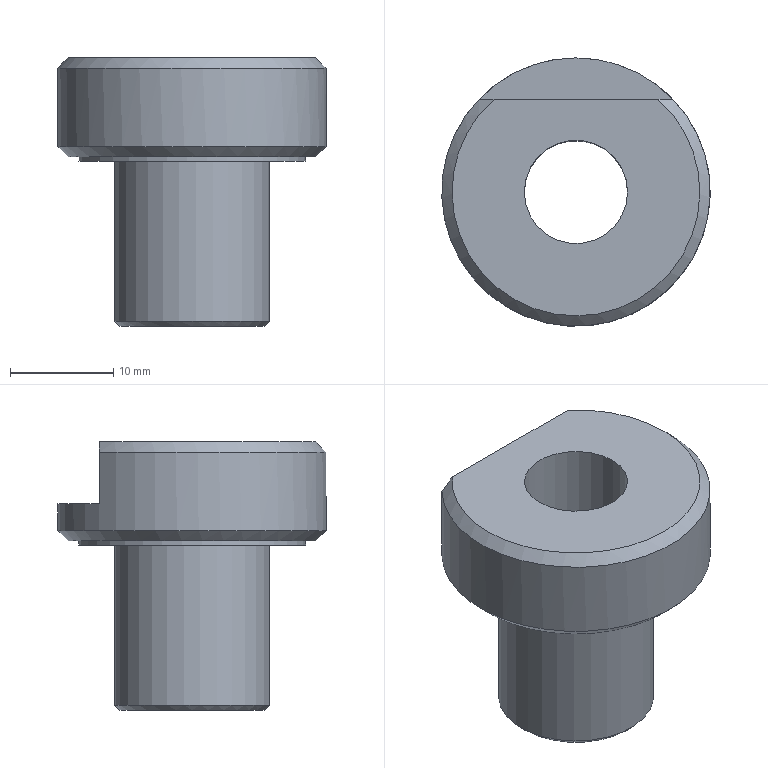Component | NX | DRILL_BUSHING | 1 solid | 13 faces | box 26 x 26 x 26 mm | volume 5648 mm3 | plane 6 | cylinder 4 | cone 3 | commonest cylinder face diameters 15 x1 22 x1 26 x1 10 x1
STEP:
#1=CARTESIAN_POINT('',(0.,0.,0.));
#2=DIRECTION('',(0.,0.,1.));
#3=DIRECTION('',(1.,0.,0.));
#4=AXIS2_PLACEMENT_3D('',#1,#2,#3);
#5=CARTESIAN_POINT('',(7.5,30.,-103.5));
#6=VERTEX_POINT('',#5);
#7=CARTESIAN_POINT('',(-0.,30.,-103.5));
#8=DIRECTION('',(0.,0.,1.));
#9=DIRECTION('',(1.,0.,0.));
#10=AXIS2_PLACEMENT_3D('',#7,#8,#9);
#11=CIRCLE('',#10,7.5);
#12=CARTESIAN_POINT('',(-0.,30.,-88.));
#13=DIRECTION('',(0.,0.,-1.));
#14=DIRECTION('',(-1.,0.,0.));
#15=AXIS2_PLACEMENT_3D('',#12,#13,#14);
#16=CYLINDRICAL_SURFACE('',#15,7.5);
#17=CARTESIAN_POINT('',(9.425,15.5));
#18=DIRECTION('',(-1.,0.));
#19=VECTOR('',#18,1.);
#20=LINE('',#17,#19);
#21=(GEOMETRIC_REPRESENTATION_CONTEXT(2)PARAMETRIC_REPRESENTATION_CONTEXT()REPRESENTATION_CONTEXT('',''));
#22=DEFINITIONAL_REPRESENTATION('',(#20),#21);
#23=PCURVE('',#16,#22);
#24=CARTESIAN_POINT('',(-0.,30.,-103.5));
#25=DIRECTION('',(0.,0.,1.));
#26=DIRECTION('',(1.,0.,0.));
#27=AXIS2_PLACEMENT_3D('',#24,#25,#26);
#28=CONICAL_SURFACE('',#27,7.5,0.7854);
#29=CARTESIAN_POINT('',(0.,0.));
#30=DIRECTION('',(1.,0.));
#31=VECTOR('',#30,1.);
#32=LINE('',#29,#31);
#33=(GEOMETRIC_REPRESENTATION_CONTEXT(2)PARAMETRIC_REPRESENTATION_CONTEXT()REPRESENTATION_CONTEXT('',''));
#34=DEFINITIONAL_REPRESENTATION('',(#32),#33);
#35=PCURVE('',#28,#34);
#36=SURFACE_CURVE('',#11,(#23,#35),.PCURVE_S1.);
#37=EDGE_CURVE('',#6,#6,#36,.T.);
#38=ORIENTED_EDGE('',*,*,#37,.T.);
#39=CARTESIAN_POINT('',(7.5,30.,-88.));
#40=VERTEX_POINT('',#39);
#41=CARTESIAN_POINT('',(7.5,30.,-88.));
#42=CARTESIAN_POINT('',(7.5,30.,-103.5));
#43=B_SPLINE_CURVE_WITH_KNOTS('',1,(#41,#42),.UNSPECIFIED.,.F.,.F.,(2,2),(0.,15.5),.PIECEWISE_BEZIER_KNOTS.);
#44=CARTESIAN_POINT('',(3.142,0.));
#45=DIRECTION('',(0.,1.));
#46=VECTOR('',#45,1.);
#47=LINE('',#44,#46);
#48=(GEOMETRIC_REPRESENTATION_CONTEXT(2)PARAMETRIC_REPRESENTATION_CONTEXT()REPRESENTATION_CONTEXT('',''));
#49=DEFINITIONAL_REPRESENTATION('',(#47),#48);
#50=PCURVE('',#16,#49);
#51=CARTESIAN_POINT('',(9.425,0.));
#52=DIRECTION('',(0.,1.));
#53=VECTOR('',#52,1.);
#54=LINE('',#51,#53);
#55=(GEOMETRIC_REPRESENTATION_CONTEXT(2)PARAMETRIC_REPRESENTATION_CONTEXT()REPRESENTATION_CONTEXT('',''));
#56=DEFINITIONAL_REPRESENTATION('',(#54),#55);
#57=PCURVE('',#16,#56);
#58=SEAM_CURVE('',#43,(#50,#57),.PCURVE_S1.);
#59=EDGE_CURVE('',#40,#6,#58,.T.);
#60=ORIENTED_EDGE('',*,*,#59,.F.);
#61=CARTESIAN_POINT('',(-0.,30.,-88.));
#62=DIRECTION('',(0.,0.,1.));
#63=DIRECTION('',(1.,0.,0.));
#64=AXIS2_PLACEMENT_3D('',#61,#62,#63);
#65=CIRCLE('',#64,7.5);
#66=CARTESIAN_POINT('',(9.425,0.));
#67=DIRECTION('',(-1.,0.));
#68=VECTOR('',#67,1.);
#69=LINE('',#66,#68);
#70=(GEOMETRIC_REPRESENTATION_CONTEXT(2)PARAMETRIC_REPRESENTATION_CONTEXT()REPRESENTATION_CONTEXT('',''));
#71=DEFINITIONAL_REPRESENTATION('',(#69),#70);
#72=PCURVE('',#16,#71);
#73=CARTESIAN_POINT('',(-0.,30.,-88.));
#74=DIRECTION('',(0.,0.,1.));
#75=DIRECTION('',(1.,0.,0.));
#76=AXIS2_PLACEMENT_3D('',#73,#74,#75);
#77=PLANE('',#76);
#78=CARTESIAN_POINT('',(0.,0.));
#79=DIRECTION('',(1.,0.));
#80=AXIS2_PLACEMENT_2D('',#78,#79);
#81=CIRCLE('',#80,7.5);
#82=(GEOMETRIC_REPRESENTATION_CONTEXT(2)PARAMETRIC_REPRESENTATION_CONTEXT()REPRESENTATION_CONTEXT('',''));
#83=DEFINITIONAL_REPRESENTATION('',(#81),#82);
#84=PCURVE('',#77,#83);
#85=SURFACE_CURVE('',#65,(#72,#84),.PCURVE_S1.);
#86=EDGE_CURVE('',#40,#40,#85,.T.);
#87=ORIENTED_EDGE('',*,*,#86,.F.);
#88=ORIENTED_EDGE('',*,*,#59,.T.);
#89=EDGE_LOOP('',(#38,#60,#87,#88));
#90=FACE_BOUND('',#89,.T.);
#91=ADVANCED_FACE('',(#90),#16,.T.);
#92=CARTESIAN_POINT('',(7.,30.,-104.));
#93=VERTEX_POINT('',#92);
#94=CARTESIAN_POINT('',(-0.,30.,-104.));
#95=DIRECTION('',(0.,0.,-1.));
#96=DIRECTION('',(1.,0.,0.));
#97=AXIS2_PLACEMENT_3D('',#94,#95,#96);
#98=CIRCLE('',#97,7.);
#99=CARTESIAN_POINT('',(-0.,30.,-104.));
#100=DIRECTION('',(0.,0.,1.));
#101=DIRECTION('',(1.,0.,0.));
#102=AXIS2_PLACEMENT_3D('',#99,#100,#101);
#103=PLANE('',#102);
#104=CARTESIAN_POINT('',(7.,0.));
#105=CARTESIAN_POINT('',(7.,-12.124));
#106=CARTESIAN_POINT('',(-3.5,-6.062));
#107=CARTESIAN_POINT('',(-14.,-0.));
#108=CARTESIAN_POINT('',(-3.5,6.062));
#109=CARTESIAN_POINT('',(7.,12.124));
#110=CARTESIAN_POINT('',(7.,0.));
#111=(BOUNDED_CURVE()B_SPLINE_CURVE(2,(#104,#105,#106,#107,#108,#109,#110),.UNSPECIFIED.,.T.,.F.)B_SPLINE_CURVE_WITH_KNOTS((1,2,2,2,2,1),(-2.094,0.,2.094,4.189,6.283,8.378),.UNSPECIFIED.)CURVE()GEOMETRIC_REPRESENTATION_ITEM()RATIONAL_B_SPLINE_CURVE((1.,0.5,1.,0.5,1.,0.5,1.))REPRESENTATION_ITEM(''));
#112=(GEOMETRIC_REPRESENTATION_CONTEXT(2)PARAMETRIC_REPRESENTATION_CONTEXT()REPRESENTATION_CONTEXT('',''));
#113=DEFINITIONAL_REPRESENTATION('',(#111),#112);
#114=PCURVE('',#103,#113);
#115=CARTESIAN_POINT('',(6.283,-0.5));
#116=DIRECTION('',(-1.,0.));
#117=VECTOR('',#116,1.);
#118=LINE('',#115,#117);
#119=(GEOMETRIC_REPRESENTATION_CONTEXT(2)PARAMETRIC_REPRESENTATION_CONTEXT()REPRESENTATION_CONTEXT('',''));
#120=DEFINITIONAL_REPRESENTATION('',(#118),#119);
#121=PCURVE('',#28,#120);
#122=SURFACE_CURVE('',#98,(#114,#121),.PCURVE_S1.);
#123=EDGE_CURVE('',#93,#93,#122,.T.);
#124=ORIENTED_EDGE('',*,*,#123,.T.);
#125=EDGE_LOOP('',(#124));
#126=FACE_BOUND('',#125,.T.);
#127=CARTESIAN_POINT('',(5.,30.,-104.));
#128=VERTEX_POINT('',#127);
#129=CARTESIAN_POINT('',(-5.,30.,-104.));
#130=VERTEX_POINT('',#129);
#131=CARTESIAN_POINT('',(-0.,30.,-104.));
#132=DIRECTION('',(0.,0.,1.));
#133=DIRECTION('',(1.,0.,0.));
#134=AXIS2_PLACEMENT_3D('',#131,#132,#133);
#135=CIRCLE('',#134,5.);
#136=CARTESIAN_POINT('',(0.,0.));
#137=DIRECTION('',(1.,0.));
#138=AXIS2_PLACEMENT_2D('',#136,#137);
#139=CIRCLE('',#138,5.);
#140=(GEOMETRIC_REPRESENTATION_CONTEXT(2)PARAMETRIC_REPRESENTATION_CONTEXT()REPRESENTATION_CONTEXT('',''));
#141=DEFINITIONAL_REPRESENTATION('',(#139),#140);
#142=PCURVE('',#103,#141);
#143=CARTESIAN_POINT('',(-0.,30.,-78.));
#144=DIRECTION('',(0.,0.,-1.));
#145=DIRECTION('',(-1.,0.,0.));
#146=AXIS2_PLACEMENT_3D('',#143,#144,#145);
#147=CYLINDRICAL_SURFACE('',#146,5.);
#148=CARTESIAN_POINT('',(3.142,26.));
#149=DIRECTION('',(-1.,0.));
#150=VECTOR('',#149,1.);
#151=LINE('',#148,#150);
#152=(GEOMETRIC_REPRESENTATION_CONTEXT(2)PARAMETRIC_REPRESENTATION_CONTEXT()REPRESENTATION_CONTEXT('',''));
#153=DEFINITIONAL_REPRESENTATION('',(#151),#152);
#154=PCURVE('',#147,#153);
#155=SURFACE_CURVE('',#135,(#142,#154),.PCURVE_S1.);
#156=EDGE_CURVE('',#128,#130,#155,.T.);
#157=ORIENTED_EDGE('',*,*,#156,.T.);
#158=CARTESIAN_POINT('',(-0.,30.,-104.));
#159=DIRECTION('',(0.,0.,1.));
#160=DIRECTION('',(1.,0.,0.));
#161=AXIS2_PLACEMENT_3D('',#158,#159,#160);
#162=CIRCLE('',#161,5.);
#163=CARTESIAN_POINT('',(0.,0.));
#164=DIRECTION('',(1.,0.));
#165=AXIS2_PLACEMENT_2D('',#163,#164);
#166=CIRCLE('',#165,5.);
#167=(GEOMETRIC_REPRESENTATION_CONTEXT(2)PARAMETRIC_REPRESENTATION_CONTEXT()REPRESENTATION_CONTEXT('',''));
#168=DEFINITIONAL_REPRESENTATION('',(#166),#167);
#169=PCURVE('',#103,#168);
#170=CARTESIAN_POINT('',(9.425,26.));
#171=DIRECTION('',(-1.,0.));
#172=VECTOR('',#171,1.);
#173=LINE('',#170,#172);
#174=(GEOMETRIC_REPRESENTATION_CONTEXT(2)PARAMETRIC_REPRESENTATION_CONTEXT()REPRESENTATION_CONTEXT('',''));
#175=DEFINITIONAL_REPRESENTATION('',(#173),#174);
#176=PCURVE('',#147,#175);
#177=SURFACE_CURVE('',#162,(#169,#176),.PCURVE_S1.);
#178=EDGE_CURVE('',#130,#128,#177,.T.);
#179=ORIENTED_EDGE('',*,*,#178,.T.);
#180=EDGE_LOOP('',(#157,#179));
#181=FACE_BOUND('',#180,.T.);
#182=ADVANCED_FACE('',(#126,#181),#103,.F.);
#183=CARTESIAN_POINT('',(11.,30.,-87.6));
#184=VERTEX_POINT('',#183);
#185=CARTESIAN_POINT('',(-0.,30.,-87.6));
#186=DIRECTION('',(0.,0.,1.));
#187=DIRECTION('',(1.,0.,0.));
#188=AXIS2_PLACEMENT_3D('',#185,#186,#187);
#189=CIRCLE('',#188,11.);
#190=CARTESIAN_POINT('',(-0.,30.,-87.6));
#191=DIRECTION('',(0.,0.,-1.));
#192=DIRECTION('',(-1.,0.,0.));
#193=AXIS2_PLACEMENT_3D('',#190,#191,#192);
#194=CYLINDRICAL_SURFACE('',#193,11.);
#195=CARTESIAN_POINT('',(9.425,0.));
#196=DIRECTION('',(-1.,0.));
#197=VECTOR('',#196,1.);
#198=LINE('',#195,#197);
#199=(GEOMETRIC_REPRESENTATION_CONTEXT(2)PARAMETRIC_REPRESENTATION_CONTEXT()REPRESENTATION_CONTEXT('',''));
#200=DEFINITIONAL_REPRESENTATION('',(#198),#199);
#201=PCURVE('',#194,#200);
#202=CARTESIAN_POINT('',(-0.,30.,-87.6));
#203=DIRECTION('',(0.,0.,1.));
#204=DIRECTION('',(1.,0.,0.));
#205=AXIS2_PLACEMENT_3D('',#202,#203,#204);
#206=PLANE('',#205);
#207=CARTESIAN_POINT('',(0.,0.));
#208=DIRECTION('',(1.,0.));
#209=AXIS2_PLACEMENT_2D('',#207,#208);
#210=CIRCLE('',#209,11.);
#211=(GEOMETRIC_REPRESENTATION_CONTEXT(2)PARAMETRIC_REPRESENTATION_CONTEXT()REPRESENTATION_CONTEXT('',''));
#212=DEFINITIONAL_REPRESENTATION('',(#210),#211);
#213=PCURVE('',#206,#212);
#214=SURFACE_CURVE('',#189,(#201,#213),.PCURVE_S1.);
#215=EDGE_CURVE('',#184,#184,#214,.T.);
#216=ORIENTED_EDGE('',*,*,#215,.F.);
#217=CARTESIAN_POINT('',(11.,30.,-88.));
#218=VERTEX_POINT('',#217);
#219=CARTESIAN_POINT('',(11.,30.,-87.6));
#220=CARTESIAN_POINT('',(11.,30.,-88.));
#221=B_SPLINE_CURVE_WITH_KNOTS('',1,(#219,#220),.UNSPECIFIED.,.F.,.F.,(2,2),(0.,0.4),.PIECEWISE_BEZIER_KNOTS.);
#222=CARTESIAN_POINT('',(9.425,0.));
#223=DIRECTION('',(0.,1.));
#224=VECTOR('',#223,1.);
#225=LINE('',#222,#224);
#226=(GEOMETRIC_REPRESENTATION_CONTEXT(2)PARAMETRIC_REPRESENTATION_CONTEXT()REPRESENTATION_CONTEXT('',''));
#227=DEFINITIONAL_REPRESENTATION('',(#225),#226);
#228=PCURVE('',#194,#227);
#229=CARTESIAN_POINT('',(3.142,0.));
#230=DIRECTION('',(0.,1.));
#231=VECTOR('',#230,1.);
#232=LINE('',#229,#231);
#233=(GEOMETRIC_REPRESENTATION_CONTEXT(2)PARAMETRIC_REPRESENTATION_CONTEXT()REPRESENTATION_CONTEXT('',''));
#234=DEFINITIONAL_REPRESENTATION('',(#232),#233);
#235=PCURVE('',#194,#234);
#236=SEAM_CURVE('',#221,(#228,#235),.PCURVE_S1.);
#237=EDGE_CURVE('',#184,#218,#236,.T.);
#238=ORIENTED_EDGE('',*,*,#237,.T.);
#239=CARTESIAN_POINT('',(-0.,30.,-88.));
#240=DIRECTION('',(0.,0.,1.));
#241=DIRECTION('',(1.,0.,0.));
#242=AXIS2_PLACEMENT_3D('',#239,#240,#241);
#243=CIRCLE('',#242,11.);
#244=CARTESIAN_POINT('',(9.425,0.4));
#245=DIRECTION('',(-1.,0.));
#246=VECTOR('',#245,1.);
#247=LINE('',#244,#246);
#248=(GEOMETRIC_REPRESENTATION_CONTEXT(2)PARAMETRIC_REPRESENTATION_CONTEXT()REPRESENTATION_CONTEXT('',''));
#249=DEFINITIONAL_REPRESENTATION('',(#247),#248);
#250=PCURVE('',#194,#249);
#251=CARTESIAN_POINT('',(0.,0.));
#252=DIRECTION('',(1.,0.));
#253=AXIS2_PLACEMENT_2D('',#251,#252);
#254=CIRCLE('',#253,11.);
#255=(GEOMETRIC_REPRESENTATION_CONTEXT(2)PARAMETRIC_REPRESENTATION_CONTEXT()REPRESENTATION_CONTEXT('',''));
#256=DEFINITIONAL_REPRESENTATION('',(#254),#255);
#257=PCURVE('',#77,#256);
#258=SURFACE_CURVE('',#243,(#250,#257),.PCURVE_S1.);
#259=EDGE_CURVE('',#218,#218,#258,.T.);
#260=ORIENTED_EDGE('',*,*,#259,.T.);
#261=ORIENTED_EDGE('',*,*,#237,.F.);
#262=EDGE_LOOP('',(#216,#238,#260,#261));
#263=FACE_BOUND('',#262,.T.);
#264=ADVANCED_FACE('',(#263),#194,.T.);
#265=ORIENTED_EDGE('',*,*,#86,.T.);
#266=EDGE_LOOP('',(#265));
#267=FACE_BOUND('',#266,.T.);
#268=ORIENTED_EDGE('',*,*,#259,.F.);
#269=EDGE_LOOP('',(#268));
#270=FACE_BOUND('',#269,.T.);
#271=ADVANCED_FACE('',(#267,#270),#77,.F.);
#272=CARTESIAN_POINT('',(13.,30.,-86.6));
#273=VERTEX_POINT('',#272);
#274=CARTESIAN_POINT('',(-9.381,39.,-86.6));
#275=VERTEX_POINT('',#274);
#276=CARTESIAN_POINT('',(-0.,30.,-86.6));
#277=DIRECTION('',(0.,0.,1.));
#278=DIRECTION('',(1.,0.,0.));
#279=AXIS2_PLACEMENT_3D('',#276,#277,#278);
#280=CIRCLE('',#279,13.);
#281=CARTESIAN_POINT('',(-0.,30.,-78.));
#282=DIRECTION('',(0.,0.,-1.));
#283=DIRECTION('',(-1.,0.,0.));
#284=AXIS2_PLACEMENT_3D('',#281,#282,#283);
#285=CYLINDRICAL_SURFACE('',#284,13.);
#286=CARTESIAN_POINT('',(3.142,8.6));
#287=DIRECTION('',(-1.,0.));
#288=VECTOR('',#287,1.);
#289=LINE('',#286,#288);
#290=(GEOMETRIC_REPRESENTATION_CONTEXT(2)PARAMETRIC_REPRESENTATION_CONTEXT()REPRESENTATION_CONTEXT('',''));
#291=DEFINITIONAL_REPRESENTATION('',(#289),#290);
#292=PCURVE('',#285,#291);
#293=CARTESIAN_POINT('',(-0.,30.,-86.6));
#294=DIRECTION('',(0.,0.,1.));
#295=DIRECTION('',(1.,0.,0.));
#296=AXIS2_PLACEMENT_3D('',#293,#294,#295);
#297=CONICAL_SURFACE('',#296,13.,0.7854);
#298=CARTESIAN_POINT('',(0.,0.));
#299=DIRECTION('',(1.,0.));
#300=VECTOR('',#299,1.);
#301=LINE('',#298,#300);
#302=(GEOMETRIC_REPRESENTATION_CONTEXT(2)PARAMETRIC_REPRESENTATION_CONTEXT()REPRESENTATION_CONTEXT('',''));
#303=DEFINITIONAL_REPRESENTATION('',(#301),#302);
#304=PCURVE('',#297,#303);
#305=SURFACE_CURVE('',#280,(#292,#304),.PCURVE_S1.);
#306=EDGE_CURVE('',#273,#275,#305,.T.);
#307=ORIENTED_EDGE('',*,*,#306,.T.);
#308=CARTESIAN_POINT('',(-9.381,39.,-84.));
#309=VERTEX_POINT('',#308);
#310=CARTESIAN_POINT('',(-9.381,39.,-84.));
#311=CARTESIAN_POINT('',(-9.381,39.,-86.6));
#312=B_SPLINE_CURVE_WITH_KNOTS('',1,(#310,#311),.UNSPECIFIED.,.F.,.F.,(2,2),(6.,8.6),.PIECEWISE_BEZIER_KNOTS.);
#313=CARTESIAN_POINT('',(0.7647,0.));
#314=DIRECTION('',(0.,1.));
#315=VECTOR('',#314,1.);
#316=LINE('',#313,#315);
#317=(GEOMETRIC_REPRESENTATION_CONTEXT(2)PARAMETRIC_REPRESENTATION_CONTEXT()REPRESENTATION_CONTEXT('',''));
#318=DEFINITIONAL_REPRESENTATION('',(#316),#317);
#319=PCURVE('',#285,#318);
#320=CARTESIAN_POINT('',(7.048,0.));
#321=DIRECTION('',(0.,1.));
#322=VECTOR('',#321,1.);
#323=LINE('',#320,#322);
#324=(GEOMETRIC_REPRESENTATION_CONTEXT(2)PARAMETRIC_REPRESENTATION_CONTEXT()REPRESENTATION_CONTEXT('',''));
#325=DEFINITIONAL_REPRESENTATION('',(#323),#324);
#326=PCURVE('',#285,#325);
#327=SEAM_CURVE('',#312,(#319,#326),.PCURVE_S1.);
#328=EDGE_CURVE('',#309,#275,#327,.T.);
#329=ORIENTED_EDGE('',*,*,#328,.F.);
#330=CARTESIAN_POINT('',(9.381,39.,-84.));
#331=VERTEX_POINT('',#330);
#332=CARTESIAN_POINT('',(-0.,30.,-84.));
#333=DIRECTION('',(0.,0.,1.));
#334=DIRECTION('',(1.,0.,0.));
#335=AXIS2_PLACEMENT_3D('',#332,#333,#334);
#336=CIRCLE('',#335,13.);
#337=CARTESIAN_POINT('',(3.142,6.));
#338=DIRECTION('',(-1.,0.));
#339=VECTOR('',#338,1.);
#340=LINE('',#337,#339);
#341=(GEOMETRIC_REPRESENTATION_CONTEXT(2)PARAMETRIC_REPRESENTATION_CONTEXT()REPRESENTATION_CONTEXT('',''));
#342=DEFINITIONAL_REPRESENTATION('',(#340),#341);
#343=PCURVE('',#285,#342);
#344=CARTESIAN_POINT('',(-0.,30.,-84.));
#345=DIRECTION('',(0.,0.,1.));
#346=DIRECTION('',(1.,0.,0.));
#347=AXIS2_PLACEMENT_3D('',#344,#345,#346);
#348=PLANE('',#347);
#349=CARTESIAN_POINT('',(0.,0.));
#350=DIRECTION('',(1.,0.));
#351=AXIS2_PLACEMENT_2D('',#349,#350);
#352=CIRCLE('',#351,13.);
#353=(GEOMETRIC_REPRESENTATION_CONTEXT(2)PARAMETRIC_REPRESENTATION_CONTEXT()REPRESENTATION_CONTEXT('',''));
#354=DEFINITIONAL_REPRESENTATION('',(#352),#353);
#355=PCURVE('',#348,#354);
#356=SURFACE_CURVE('',#336,(#343,#355),.PCURVE_S1.);
#357=EDGE_CURVE('',#331,#309,#356,.T.);
#358=ORIENTED_EDGE('',*,*,#357,.F.);
#359=CARTESIAN_POINT('',(9.381,39.,-79.));
#360=VERTEX_POINT('',#359);
#361=CARTESIAN_POINT('',(9.381,39.,-78.));
#362=DIRECTION('',(0.,0.,1.));
#363=VECTOR('',#362,1.);
#364=LINE('',#361,#363);
#365=CARTESIAN_POINT('',(2.377,0.));
#366=DIRECTION('',(0.,-1.));
#367=VECTOR('',#366,1.);
#368=LINE('',#365,#367);
#369=(GEOMETRIC_REPRESENTATION_CONTEXT(2)PARAMETRIC_REPRESENTATION_CONTEXT()REPRESENTATION_CONTEXT('',''));
#370=DEFINITIONAL_REPRESENTATION('',(#368),#369);
#371=PCURVE('',#285,#370);
#372=CARTESIAN_POINT('',(-14.5,39.,-84.));
#373=DIRECTION('',(0.,-1.,0.));
#374=DIRECTION('',(1.,0.,0.));
#375=AXIS2_PLACEMENT_3D('',#372,#373,#374);
#376=PLANE('',#375);
#377=CARTESIAN_POINT('',(23.881,6.));
#378=DIRECTION('',(0.,1.));
#379=VECTOR('',#378,1.);
#380=LINE('',#377,#379);
#381=(GEOMETRIC_REPRESENTATION_CONTEXT(2)PARAMETRIC_REPRESENTATION_CONTEXT()REPRESENTATION_CONTEXT('',''));
#382=DEFINITIONAL_REPRESENTATION('',(#380),#381);
#383=PCURVE('',#376,#382);
#384=SURFACE_CURVE('',#364,(#371,#383),.PCURVE_S1.);
#385=EDGE_CURVE('',#331,#360,#384,.T.);
#386=ORIENTED_EDGE('',*,*,#385,.T.);
#387=CARTESIAN_POINT('',(-9.381,39.,-79.));
#388=VERTEX_POINT('',#387);
#389=CARTESIAN_POINT('',(-0.,30.,-79.));
#390=DIRECTION('',(0.,0.,-1.));
#391=DIRECTION('',(1.,0.,0.));
#392=AXIS2_PLACEMENT_3D('',#389,#390,#391);
#393=CIRCLE('',#392,13.);
#394=CARTESIAN_POINT('',(-3.142,1.));
#395=DIRECTION('',(1.,0.));
#396=VECTOR('',#395,1.);
#397=LINE('',#394,#396);
#398=(GEOMETRIC_REPRESENTATION_CONTEXT(2)PARAMETRIC_REPRESENTATION_CONTEXT()REPRESENTATION_CONTEXT('',''));
#399=DEFINITIONAL_REPRESENTATION('',(#397),#398);
#400=PCURVE('',#285,#399);
#401=CARTESIAN_POINT('',(-0.,30.,-78.));
#402=DIRECTION('',(0.,0.,-1.));
#403=DIRECTION('',(-1.,0.,0.));
#404=AXIS2_PLACEMENT_3D('',#401,#402,#403);
#405=CONICAL_SURFACE('',#404,12.,0.7854);
#406=CARTESIAN_POINT('',(-3.142,1.));
#407=DIRECTION('',(1.,0.));
#408=VECTOR('',#407,1.);
#409=LINE('',#406,#408);
#410=(GEOMETRIC_REPRESENTATION_CONTEXT(2)PARAMETRIC_REPRESENTATION_CONTEXT()REPRESENTATION_CONTEXT('',''));
#411=DEFINITIONAL_REPRESENTATION('',(#409),#410);
#412=PCURVE('',#405,#411);
#413=SURFACE_CURVE('',#393,(#400,#412),.PCURVE_S1.);
#414=EDGE_CURVE('',#360,#388,#413,.T.);
#415=ORIENTED_EDGE('',*,*,#414,.T.);
#416=CARTESIAN_POINT('',(-9.381,39.,-78.));
#417=DIRECTION('',(0.,0.,-1.));
#418=VECTOR('',#417,1.);
#419=LINE('',#416,#418);
#420=CARTESIAN_POINT('',(7.048,0.));
#421=DIRECTION('',(0.,1.));
#422=VECTOR('',#421,1.);
#423=LINE('',#420,#422);
#424=(GEOMETRIC_REPRESENTATION_CONTEXT(2)PARAMETRIC_REPRESENTATION_CONTEXT()REPRESENTATION_CONTEXT('',''));
#425=DEFINITIONAL_REPRESENTATION('',(#423),#424);
#426=PCURVE('',#285,#425);
#427=CARTESIAN_POINT('',(5.119,6.));
#428=DIRECTION('',(0.,-1.));
#429=VECTOR('',#428,1.);
#430=LINE('',#427,#429);
#431=(GEOMETRIC_REPRESENTATION_CONTEXT(2)PARAMETRIC_REPRESENTATION_CONTEXT()REPRESENTATION_CONTEXT('',''));
#432=DEFINITIONAL_REPRESENTATION('',(#430),#431);
#433=PCURVE('',#376,#432);
#434=SURFACE_CURVE('',#419,(#426,#433),.PCURVE_S1.);
#435=EDGE_CURVE('',#388,#309,#434,.T.);
#436=ORIENTED_EDGE('',*,*,#435,.T.);
#437=ORIENTED_EDGE('',*,*,#328,.T.);
#438=CARTESIAN_POINT('',(-0.,30.,-86.6));
#439=DIRECTION('',(0.,0.,1.));
#440=DIRECTION('',(1.,0.,0.));
#441=AXIS2_PLACEMENT_3D('',#438,#439,#440);
#442=CIRCLE('',#441,13.);
#443=CARTESIAN_POINT('',(9.425,8.6));
#444=DIRECTION('',(-1.,0.));
#445=VECTOR('',#444,1.);
#446=LINE('',#443,#445);
#447=(GEOMETRIC_REPRESENTATION_CONTEXT(2)PARAMETRIC_REPRESENTATION_CONTEXT()REPRESENTATION_CONTEXT('',''));
#448=DEFINITIONAL_REPRESENTATION('',(#446),#447);
#449=PCURVE('',#285,#448);
#450=CARTESIAN_POINT('',(0.,0.));
#451=DIRECTION('',(1.,0.));
#452=VECTOR('',#451,1.);
#453=LINE('',#450,#452);
#454=(GEOMETRIC_REPRESENTATION_CONTEXT(2)PARAMETRIC_REPRESENTATION_CONTEXT()REPRESENTATION_CONTEXT('',''));
#455=DEFINITIONAL_REPRESENTATION('',(#453),#454);
#456=PCURVE('',#297,#455);
#457=SURFACE_CURVE('',#442,(#449,#456),.PCURVE_S1.);
#458=EDGE_CURVE('',#275,#273,#457,.T.);
#459=ORIENTED_EDGE('',*,*,#458,.T.);
#460=EDGE_LOOP('',(#307,#329,#358,#386,#415,#436,#437,#459));
#461=FACE_BOUND('',#460,.T.);
#462=ADVANCED_FACE('',(#461),#285,.T.);
#463=CARTESIAN_POINT('',(-7.937,39.,-78.));
#464=VERTEX_POINT('',#463);
#465=CARTESIAN_POINT('',(7.937,39.,-78.));
#466=VERTEX_POINT('',#465);
#467=CARTESIAN_POINT('',(-14.5,39.,-78.));
#468=DIRECTION('',(1.,0.,0.));
#469=VECTOR('',#468,1.);
#470=LINE('',#467,#469);
#471=CARTESIAN_POINT('',(-0.,30.,-78.));
#472=DIRECTION('',(0.,0.,1.));
#473=DIRECTION('',(1.,0.,0.));
#474=AXIS2_PLACEMENT_3D('',#471,#472,#473);
#475=PLANE('',#474);
#476=CARTESIAN_POINT('',(-14.5,9.));
#477=DIRECTION('',(1.,0.));
#478=VECTOR('',#477,1.);
#479=LINE('',#476,#478);
#480=(GEOMETRIC_REPRESENTATION_CONTEXT(2)PARAMETRIC_REPRESENTATION_CONTEXT()REPRESENTATION_CONTEXT('',''));
#481=DEFINITIONAL_REPRESENTATION('',(#479),#480);
#482=PCURVE('',#475,#481);
#483=CARTESIAN_POINT('',(0.,6.));
#484=DIRECTION('',(1.,0.));
#485=VECTOR('',#484,1.);
#486=LINE('',#483,#485);
#487=(GEOMETRIC_REPRESENTATION_CONTEXT(2)PARAMETRIC_REPRESENTATION_CONTEXT()REPRESENTATION_CONTEXT('',''));
#488=DEFINITIONAL_REPRESENTATION('',(#486),#487);
#489=PCURVE('',#376,#488);
#490=SURFACE_CURVE('',#470,(#482,#489),.PCURVE_S1.);
#491=EDGE_CURVE('',#464,#466,#490,.T.);
#492=ORIENTED_EDGE('',*,*,#491,.F.);
#493=CARTESIAN_POINT('',(-0.,30.,-78.));
#494=DIRECTION('',(0.,0.,1.));
#495=DIRECTION('',(1.,0.,0.));
#496=AXIS2_PLACEMENT_3D('',#493,#494,#495);
#497=CIRCLE('',#496,12.);
#498=CARTESIAN_POINT('',(0.,0.));
#499=DIRECTION('',(1.,0.));
#500=AXIS2_PLACEMENT_2D('',#498,#499);
#501=CIRCLE('',#500,12.);
#502=(GEOMETRIC_REPRESENTATION_CONTEXT(2)PARAMETRIC_REPRESENTATION_CONTEXT()REPRESENTATION_CONTEXT('',''));
#503=DEFINITIONAL_REPRESENTATION('',(#501),#502);
#504=PCURVE('',#475,#503);
#505=CARTESIAN_POINT('',(9.425,0.));
#506=DIRECTION('',(-1.,-0.));
#507=VECTOR('',#506,1.);
#508=LINE('',#505,#507);
#509=(GEOMETRIC_REPRESENTATION_CONTEXT(2)PARAMETRIC_REPRESENTATION_CONTEXT()REPRESENTATION_CONTEXT('',''));
#510=DEFINITIONAL_REPRESENTATION('',(#508),#509);
#511=PCURVE('',#405,#510);
#512=SURFACE_CURVE('',#497,(#504,#511),.PCURVE_S1.);
#513=EDGE_CURVE('',#464,#466,#512,.T.);
#514=ORIENTED_EDGE('',*,*,#513,.T.);
#515=EDGE_LOOP('',(#492,#514));
#516=FACE_BOUND('',#515,.T.);
#517=CARTESIAN_POINT('',(-5.,30.,-78.));
#518=VERTEX_POINT('',#517);
#519=CARTESIAN_POINT('',(-0.,30.,-78.));
#520=DIRECTION('',(0.,0.,-1.));
#521=DIRECTION('',(-1.,0.,0.));
#522=AXIS2_PLACEMENT_3D('',#519,#520,#521);
#523=CIRCLE('',#522,5.);
#524=CARTESIAN_POINT('',(-5.,0.));
#525=CARTESIAN_POINT('',(-5.,8.66));
#526=CARTESIAN_POINT('',(2.5,4.33));
#527=CARTESIAN_POINT('',(10.,0.));
#528=CARTESIAN_POINT('',(2.5,-4.33));
#529=CARTESIAN_POINT('',(-5.,-8.66));
#530=CARTESIAN_POINT('',(-5.,0.));
#531=(BOUNDED_CURVE()B_SPLINE_CURVE(2,(#524,#525,#526,#527,#528,#529,#530),.UNSPECIFIED.,.T.,.F.)B_SPLINE_CURVE_WITH_KNOTS((1,2,2,2,2,1),(-2.094,0.,2.094,4.189,6.283,8.378),.UNSPECIFIED.)CURVE()GEOMETRIC_REPRESENTATION_ITEM()RATIONAL_B_SPLINE_CURVE((1.,0.5,1.,0.5,1.,0.5,1.))REPRESENTATION_ITEM(''));
#532=(GEOMETRIC_REPRESENTATION_CONTEXT(2)PARAMETRIC_REPRESENTATION_CONTEXT()REPRESENTATION_CONTEXT('',''));
#533=DEFINITIONAL_REPRESENTATION('',(#531),#532);
#534=PCURVE('',#475,#533);
#535=CARTESIAN_POINT('',(0.,0.));
#536=DIRECTION('',(1.,0.));
#537=VECTOR('',#536,1.);
#538=LINE('',#535,#537);
#539=(GEOMETRIC_REPRESENTATION_CONTEXT(2)PARAMETRIC_REPRESENTATION_CONTEXT()REPRESENTATION_CONTEXT('',''));
#540=DEFINITIONAL_REPRESENTATION('',(#538),#539);
#541=PCURVE('',#147,#540);
#542=SURFACE_CURVE('',#523,(#534,#541),.PCURVE_S1.);
#543=EDGE_CURVE('',#518,#518,#542,.T.);
#544=ORIENTED_EDGE('',*,*,#543,.T.);
#545=EDGE_LOOP('',(#544));
#546=FACE_BOUND('',#545,.T.);
#547=ADVANCED_FACE('',(#516,#546),#475,.T.);
#548=CARTESIAN_POINT('',(12.,30.,-87.6));
#549=VERTEX_POINT('',#548);
#550=CARTESIAN_POINT('',(-0.,30.,-87.6));
#551=DIRECTION('',(0.,0.,-1.));
#552=DIRECTION('',(1.,0.,0.));
#553=AXIS2_PLACEMENT_3D('',#550,#551,#552);
#554=CIRCLE('',#553,12.);
#555=CARTESIAN_POINT('',(12.,0.));
#556=CARTESIAN_POINT('',(12.,-20.785));
#557=CARTESIAN_POINT('',(-6.,-10.392));
#558=CARTESIAN_POINT('',(-24.,-0.));
#559=CARTESIAN_POINT('',(-6.,10.392));
#560=CARTESIAN_POINT('',(12.,20.785));
#561=CARTESIAN_POINT('',(12.,0.));
#562=(BOUNDED_CURVE()B_SPLINE_CURVE(2,(#555,#556,#557,#558,#559,#560,#561),.UNSPECIFIED.,.T.,.F.)B_SPLINE_CURVE_WITH_KNOTS((1,2,2,2,2,1),(-2.094,0.,2.094,4.189,6.283,8.378),.UNSPECIFIED.)CURVE()GEOMETRIC_REPRESENTATION_ITEM()RATIONAL_B_SPLINE_CURVE((1.,0.5,1.,0.5,1.,0.5,1.))REPRESENTATION_ITEM(''));
#563=(GEOMETRIC_REPRESENTATION_CONTEXT(2)PARAMETRIC_REPRESENTATION_CONTEXT()REPRESENTATION_CONTEXT('',''));
#564=DEFINITIONAL_REPRESENTATION('',(#562),#563);
#565=PCURVE('',#206,#564);
#566=CARTESIAN_POINT('',(6.283,-1.));
#567=DIRECTION('',(-1.,0.));
#568=VECTOR('',#567,1.);
#569=LINE('',#566,#568);
#570=(GEOMETRIC_REPRESENTATION_CONTEXT(2)PARAMETRIC_REPRESENTATION_CONTEXT()REPRESENTATION_CONTEXT('',''));
#571=DEFINITIONAL_REPRESENTATION('',(#569),#570);
#572=PCURVE('',#297,#571);
#573=SURFACE_CURVE('',#554,(#565,#572),.PCURVE_S1.);
#574=EDGE_CURVE('',#549,#549,#573,.T.);
#575=ORIENTED_EDGE('',*,*,#574,.T.);
#576=EDGE_LOOP('',(#575));
#577=FACE_BOUND('',#576,.T.);
#578=ORIENTED_EDGE('',*,*,#215,.T.);
#579=EDGE_LOOP('',(#578));
#580=FACE_BOUND('',#579,.T.);
#581=ADVANCED_FACE('',(#577,#580),#206,.F.);
#582=ORIENTED_EDGE('',*,*,#543,.T.);
#583=CARTESIAN_POINT('',(-5.,30.,-78.));
#584=CARTESIAN_POINT('',(-5.,30.,-104.));
#585=B_SPLINE_CURVE_WITH_KNOTS('',1,(#583,#584),.UNSPECIFIED.,.F.,.F.,(2,2),(0.,26.),.PIECEWISE_BEZIER_KNOTS.);
#586=CARTESIAN_POINT('',(6.283,0.));
#587=DIRECTION('',(0.,1.));
#588=VECTOR('',#587,1.);
#589=LINE('',#586,#588);
#590=(GEOMETRIC_REPRESENTATION_CONTEXT(2)PARAMETRIC_REPRESENTATION_CONTEXT()REPRESENTATION_CONTEXT('',''));
#591=DEFINITIONAL_REPRESENTATION('',(#589),#590);
#592=PCURVE('',#147,#591);
#593=CARTESIAN_POINT('',(0.,0.));
#594=DIRECTION('',(0.,1.));
#595=VECTOR('',#594,1.);
#596=LINE('',#593,#595);
#597=(GEOMETRIC_REPRESENTATION_CONTEXT(2)PARAMETRIC_REPRESENTATION_CONTEXT()REPRESENTATION_CONTEXT('',''));
#598=DEFINITIONAL_REPRESENTATION('',(#596),#597);
#599=PCURVE('',#147,#598);
#600=SEAM_CURVE('',#585,(#592,#599),.PCURVE_S1.);
#601=EDGE_CURVE('',#518,#130,#600,.T.);
#602=ORIENTED_EDGE('',*,*,#601,.T.);
#603=ORIENTED_EDGE('',*,*,#178,.T.);
#604=ORIENTED_EDGE('',*,*,#156,.T.);
#605=ORIENTED_EDGE('',*,*,#601,.F.);
#606=EDGE_LOOP('',(#582,#602,#603,#604,#605));
#607=FACE_BOUND('',#606,.F.);
#608=ADVANCED_FACE('',(#607),#147,.F.);
#609=ORIENTED_EDGE('',*,*,#357,.T.);
#610=CARTESIAN_POINT('',(-14.5,39.,-84.));
#611=DIRECTION('',(-1.,-0.,0.));
#612=VECTOR('',#611,1.);
#613=LINE('',#610,#612);
#614=CARTESIAN_POINT('',(-14.5,9.));
#615=DIRECTION('',(-1.,-0.));
#616=VECTOR('',#615,1.);
#617=LINE('',#614,#616);
#618=(GEOMETRIC_REPRESENTATION_CONTEXT(2)PARAMETRIC_REPRESENTATION_CONTEXT()REPRESENTATION_CONTEXT('',''));
#619=DEFINITIONAL_REPRESENTATION('',(#617),#618);
#620=PCURVE('',#348,#619);
#621=CARTESIAN_POINT('',(0.,0.));
#622=DIRECTION('',(-1.,0.));
#623=VECTOR('',#622,1.);
#624=LINE('',#621,#623);
#625=(GEOMETRIC_REPRESENTATION_CONTEXT(2)PARAMETRIC_REPRESENTATION_CONTEXT()REPRESENTATION_CONTEXT('',''));
#626=DEFINITIONAL_REPRESENTATION('',(#624),#625);
#627=PCURVE('',#376,#626);
#628=SURFACE_CURVE('',#613,(#620,#627),.PCURVE_S1.);
#629=EDGE_CURVE('',#331,#309,#628,.T.);
#630=ORIENTED_EDGE('',*,*,#629,.F.);
#631=EDGE_LOOP('',(#609,#630));
#632=FACE_BOUND('',#631,.T.);
#633=ADVANCED_FACE('',(#632),#348,.T.);
#634=ORIENTED_EDGE('',*,*,#491,.T.);
#635=CARTESIAN_POINT('',(7.937,39.,-78.));
#636=CARTESIAN_POINT('',(8.425,39.,-78.323));
#637=CARTESIAN_POINT('',(8.906,39.,-78.657));
#638=CARTESIAN_POINT('',(9.381,39.,-79.));
#639=B_SPLINE_CURVE_WITH_KNOTS('',3,(#635,#636,#637,#638),.UNSPECIFIED.,.F.,.F.,(4,4),(0.,1.),.PIECEWISE_BEZIER_KNOTS.);
#640=CARTESIAN_POINT('',(22.437,6.));
#641=CARTESIAN_POINT('',(22.925,5.677));
#642=CARTESIAN_POINT('',(23.406,5.343));
#643=CARTESIAN_POINT('',(23.881,5.));
#644=B_SPLINE_CURVE_WITH_KNOTS('',3,(#640,#641,#642,#643),.UNSPECIFIED.,.F.,.F.,(4,4),(0.,1.),.PIECEWISE_BEZIER_KNOTS.);
#645=(GEOMETRIC_REPRESENTATION_CONTEXT(2)PARAMETRIC_REPRESENTATION_CONTEXT()REPRESENTATION_CONTEXT('',''));
#646=DEFINITIONAL_REPRESENTATION('',(#644),#645);
#647=PCURVE('',#376,#646);
#648=CARTESIAN_POINT('',(2.294,0.));
#649=CARTESIAN_POINT('',(2.377,1.));
#650=B_SPLINE_CURVE_WITH_KNOTS('',1,(#648,#649),.UNSPECIFIED.,.F.,.F.,(2,2),(0.,1.),.PIECEWISE_BEZIER_KNOTS.);
#651=(GEOMETRIC_REPRESENTATION_CONTEXT(2)PARAMETRIC_REPRESENTATION_CONTEXT()REPRESENTATION_CONTEXT('',''));
#652=DEFINITIONAL_REPRESENTATION('',(#650),#651);
#653=PCURVE('',#405,#652);
#654=SURFACE_CURVE('',#639,(#647,#653),.PCURVE_S1.);
#655=EDGE_CURVE('',#466,#360,#654,.T.);
#656=ORIENTED_EDGE('',*,*,#655,.T.);
#657=ORIENTED_EDGE('',*,*,#385,.F.);
#658=ORIENTED_EDGE('',*,*,#629,.T.);
#659=ORIENTED_EDGE('',*,*,#435,.F.);
#660=CARTESIAN_POINT('',(-9.381,39.,-79.));
#661=CARTESIAN_POINT('',(-8.906,39.,-78.657));
#662=CARTESIAN_POINT('',(-8.425,39.,-78.323));
#663=CARTESIAN_POINT('',(-7.937,39.,-78.));
#664=B_SPLINE_CURVE_WITH_KNOTS('',3,(#660,#661,#662,#663),.UNSPECIFIED.,.F.,.F.,(4,4),(0.,1.),.PIECEWISE_BEZIER_KNOTS.);
#665=CARTESIAN_POINT('',(5.119,5.));
#666=CARTESIAN_POINT('',(5.594,5.343));
#667=CARTESIAN_POINT('',(6.075,5.677));
#668=CARTESIAN_POINT('',(6.563,6.));
#669=B_SPLINE_CURVE_WITH_KNOTS('',3,(#665,#666,#667,#668),.UNSPECIFIED.,.F.,.F.,(4,4),(0.,1.),.PIECEWISE_BEZIER_KNOTS.);
#670=(GEOMETRIC_REPRESENTATION_CONTEXT(2)PARAMETRIC_REPRESENTATION_CONTEXT()REPRESENTATION_CONTEXT('',''));
#671=DEFINITIONAL_REPRESENTATION('',(#669),#670);
#672=PCURVE('',#376,#671);
#673=CARTESIAN_POINT('',(7.048,1.));
#674=CARTESIAN_POINT('',(7.131,0.));
#675=B_SPLINE_CURVE_WITH_KNOTS('',1,(#673,#674),.UNSPECIFIED.,.F.,.F.,(2,2),(0.,1.),.PIECEWISE_BEZIER_KNOTS.);
#676=(GEOMETRIC_REPRESENTATION_CONTEXT(2)PARAMETRIC_REPRESENTATION_CONTEXT()REPRESENTATION_CONTEXT('',''));
#677=DEFINITIONAL_REPRESENTATION('',(#675),#676);
#678=PCURVE('',#405,#677);
#679=SURFACE_CURVE('',#664,(#672,#678),.PCURVE_S1.);
#680=EDGE_CURVE('',#388,#464,#679,.T.);
#681=ORIENTED_EDGE('',*,*,#680,.T.);
#682=EDGE_LOOP('',(#634,#656,#657,#658,#659,#681));
#683=FACE_BOUND('',#682,.T.);
#684=ADVANCED_FACE('',(#683),#376,.F.);
#685=ORIENTED_EDGE('',*,*,#574,.F.);
#686=CARTESIAN_POINT('',(12.,30.,-87.6));
#687=CARTESIAN_POINT('',(13.,30.,-86.6));
#688=B_SPLINE_CURVE_WITH_KNOTS('',1,(#686,#687),.UNSPECIFIED.,.F.,.F.,(2,2),(-1.414,0.),.PIECEWISE_BEZIER_KNOTS.);
#689=CARTESIAN_POINT('',(6.283,0.));
#690=DIRECTION('',(0.,1.));
#691=VECTOR('',#690,1.);
#692=LINE('',#689,#691);
#693=(GEOMETRIC_REPRESENTATION_CONTEXT(2)PARAMETRIC_REPRESENTATION_CONTEXT()REPRESENTATION_CONTEXT('',''));
#694=DEFINITIONAL_REPRESENTATION('',(#692),#693);
#695=PCURVE('',#297,#694);
#696=CARTESIAN_POINT('',(0.,0.));
#697=DIRECTION('',(0.,1.));
#698=VECTOR('',#697,1.);
#699=LINE('',#696,#698);
#700=(GEOMETRIC_REPRESENTATION_CONTEXT(2)PARAMETRIC_REPRESENTATION_CONTEXT()REPRESENTATION_CONTEXT('',''));
#701=DEFINITIONAL_REPRESENTATION('',(#699),#700);
#702=PCURVE('',#297,#701);
#703=SEAM_CURVE('',#688,(#695,#702),.PCURVE_S1.);
#704=EDGE_CURVE('',#549,#273,#703,.T.);
#705=ORIENTED_EDGE('',*,*,#704,.T.);
#706=ORIENTED_EDGE('',*,*,#458,.F.);
#707=ORIENTED_EDGE('',*,*,#306,.F.);
#708=ORIENTED_EDGE('',*,*,#704,.F.);
#709=EDGE_LOOP('',(#685,#705,#706,#707,#708));
#710=FACE_BOUND('',#709,.T.);
#711=ADVANCED_FACE('',(#710),#297,.T.);
#712=ORIENTED_EDGE('',*,*,#680,.F.);
#713=ORIENTED_EDGE('',*,*,#414,.F.);
#714=ORIENTED_EDGE('',*,*,#655,.F.);
#715=ORIENTED_EDGE('',*,*,#513,.F.);
#716=EDGE_LOOP('',(#712,#713,#714,#715));
#717=FACE_BOUND('',#716,.T.);
#718=ADVANCED_FACE('',(#717),#405,.T.);
#719=ORIENTED_EDGE('',*,*,#123,.F.);
#720=CARTESIAN_POINT('',(7.,30.,-104.));
#721=CARTESIAN_POINT('',(7.5,30.,-103.5));
#722=B_SPLINE_CURVE_WITH_KNOTS('',1,(#720,#721),.UNSPECIFIED.,.F.,.F.,(2,2),(-0.7071,0.),.PIECEWISE_BEZIER_KNOTS.);
#723=CARTESIAN_POINT('',(6.283,0.));
#724=DIRECTION('',(0.,1.));
#725=VECTOR('',#724,1.);
#726=LINE('',#723,#725);
#727=(GEOMETRIC_REPRESENTATION_CONTEXT(2)PARAMETRIC_REPRESENTATION_CONTEXT()REPRESENTATION_CONTEXT('',''));
#728=DEFINITIONAL_REPRESENTATION('',(#726),#727);
#729=PCURVE('',#28,#728);
#730=CARTESIAN_POINT('',(0.,0.));
#731=DIRECTION('',(0.,1.));
#732=VECTOR('',#731,1.);
#733=LINE('',#730,#732);
#734=(GEOMETRIC_REPRESENTATION_CONTEXT(2)PARAMETRIC_REPRESENTATION_CONTEXT()REPRESENTATION_CONTEXT('',''));
#735=DEFINITIONAL_REPRESENTATION('',(#733),#734);
#736=PCURVE('',#28,#735);
#737=SEAM_CURVE('',#722,(#729,#736),.PCURVE_S1.);
#738=EDGE_CURVE('',#93,#6,#737,.T.);
#739=ORIENTED_EDGE('',*,*,#738,.T.);
#740=ORIENTED_EDGE('',*,*,#37,.F.);
#741=ORIENTED_EDGE('',*,*,#738,.F.);
#742=EDGE_LOOP('',(#719,#739,#740,#741));
#743=FACE_BOUND('',#742,.T.);
#744=ADVANCED_FACE('',(#743),#28,.T.);
#745=CLOSED_SHELL('',(#91,#182,#264,#271,#462,#547,#581,#608,#633,#684,#711,#718,#744));
#746=MANIFOLD_SOLID_BREP('',#745);
#747=(LENGTH_UNIT()NAMED_UNIT(*)SI_UNIT(.MILLI.,.METRE.));
#748=UNCERTAINTY_MEASURE_WITH_UNIT(LENGTH_MEASURE(0.005),#747,'','');
#749=(NAMED_UNIT(*)PLANE_ANGLE_UNIT()SI_UNIT($,.RADIAN.));
#750=(NAMED_UNIT(*)SI_UNIT($,.STERADIAN.)SOLID_ANGLE_UNIT());
#751=(GEOMETRIC_REPRESENTATION_CONTEXT(3)GLOBAL_UNCERTAINTY_ASSIGNED_CONTEXT((#748))GLOBAL_UNIT_ASSIGNED_CONTEXT((#747,#749,#750))REPRESENTATION_CONTEXT('',''));
#752=ADVANCED_BREP_SHAPE_REPRESENTATION('',(#4,#746),#751);